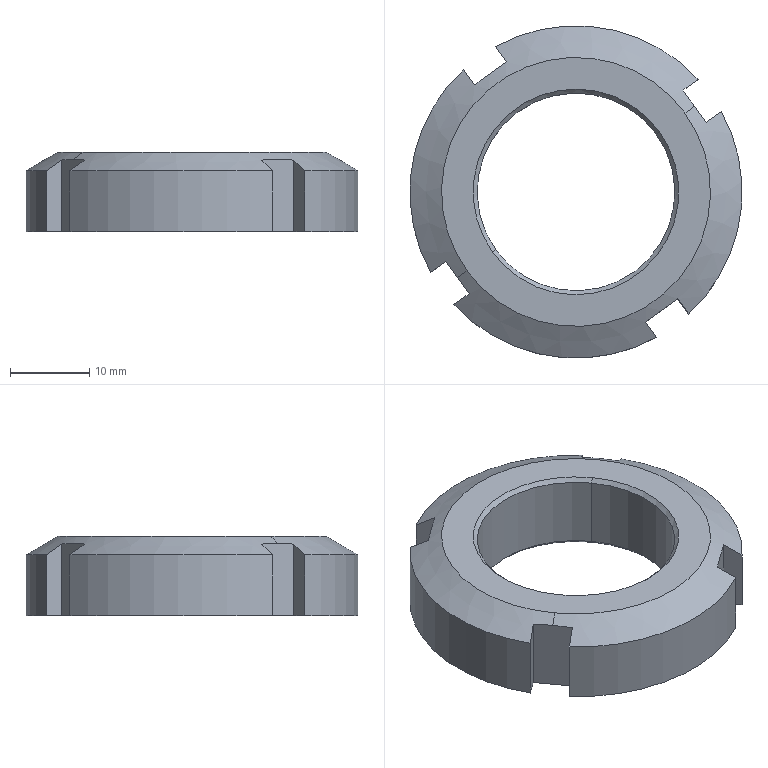Component | SolidWorks | M25_1.5RoundNut(GB-T812-1988)0-2 | 1 solid | 26 faces | box 42 x 42 x 10 mm | volume 7943 mm3 | plane 14 | cone 6 | cylinder 6 | commonest cylinder face diameters 42 x4 25 x2
build123d program:
from build123d import *

# Parameters (mm, degrees)
SKETCH2_W          = 5
SKETCH2_H          = 4.32
SKETCH2_W_2        = 4.32
SKETCH2_H_2        = 5
CUT_EXTRUDE1_DEPTH = 32.337


with BuildPart() as part:
    # Sketch1 → Revolve1 (revolve)
    with BuildSketch(Plane.XY, mode=Mode.PRIVATE) as revolve1_sk:
        Polygon((17, 5), (21, 2.69), (21, -5), (13, -5), (12.5, -4.5), (12.5, 4.5), (13, 5), align=None)
    revolve(revolve1_sk.sketch.rotate(Axis((0, 38.731, 0), (0, -1, 0)), 90), axis=Axis((0, 38.731, 0), (0, -1, 0)))

    # Sketch2 → Cut-Extrude1 (cut, through all)
    with BuildSketch(Plane(origin=(0, 5, 0), x_dir=(1, 0, 0), z_dir=(0, 1, 0))):
        with Locations((0, 20.66)):
            Rectangle(SKETCH2_W, SKETCH2_H)
        with Locations((20.66, 0)):
            Rectangle(SKETCH2_W_2, SKETCH2_H_2)
        with Locations((0, -20.66)):
            Rectangle(SKETCH2_W, SKETCH2_H)
        with Locations((-20.66, 0)):
            Rectangle(SKETCH2_W_2, SKETCH2_H_2)
    extrude(amount=-CUT_EXTRUDE1_DEPTH, mode=Mode.SUBTRACT)


solid = part.part

# Placed as in the assembly
solid = solid.moved(Location((-15.093, -37.782, 199.255), (-90, -35.881, -180)))
STEP:
#1=COLOUR_RGB('',0.7922,0.8196,0.9333);
#2=FILL_AREA_STYLE_COLOUR('',#1);
#3=FILL_AREA_STYLE('',(#2));
#4=SURFACE_STYLE_FILL_AREA(#3);
#5=SURFACE_SIDE_STYLE('',(#4));
#6=SURFACE_STYLE_USAGE(.BOTH.,#5);
#7=PRESENTATION_STYLE_ASSIGNMENT((#6));
#8=CARTESIAN_POINT('',(-0.1955,-1.199,7.668));
#9=VERTEX_POINT('',#8);
#10=CARTESIAN_POINT('',(-0.993,-1.776,7.668));
#11=VERTEX_POINT('',#10);
#12=CARTESIAN_POINT('',(-0.5942,-1.487,7.668));
#13=DIRECTION('',(0.,0.,1.));
#14=DIRECTION('',(-0.8102,-0.5861,0.));
#15=AXIS2_PLACEMENT_3D('',#12,#13,#14);
#16=CIRCLE('',#15,0.4921);
#17=EDGE_CURVE('',#9,#11,#16,.T.);
#18=ORIENTED_EDGE('',*,*,#17,.T.);
#19=CARTESIAN_POINT('',(-1.009,-1.787,7.648));
#20=VERTEX_POINT('',#19);
#21=CARTESIAN_POINT('',(-0.993,-1.776,7.668));
#22=DIRECTION('',(-0.5729,-0.4144,-0.7071));
#23=VECTOR('',#22,39.37);
#24=LINE('',#21,#23);
#25=EDGE_CURVE('',#11,#20,#24,.T.);
#26=ORIENTED_EDGE('',*,*,#25,.T.);
#27=CARTESIAN_POINT('',(-0.1795,-1.187,7.648));
#28=VERTEX_POINT('',#27);
#29=CARTESIAN_POINT('',(-0.5942,-1.487,7.648));
#30=DIRECTION('',(0.,0.,1.));
#31=DIRECTION('',(-0.8102,-0.5861,0.));
#32=AXIS2_PLACEMENT_3D('',#29,#30,#31);
#33=CIRCLE('',#32,0.5118);
#34=EDGE_CURVE('',#28,#20,#33,.T.);
#35=ORIENTED_EDGE('',*,*,#34,.F.);
#36=CARTESIAN_POINT('',(-0.1955,-1.199,7.668));
#37=DIRECTION('',(0.5729,0.4144,-0.7071));
#38=VECTOR('',#37,39.37);
#39=LINE('',#36,#38);
#40=EDGE_CURVE('',#9,#28,#39,.T.);
#41=ORIENTED_EDGE('',*,*,#40,.F.);
#42=EDGE_LOOP('',(#18,#26,#35,#41));
#43=FACE_OUTER_BOUND('',#42,.T.);
#44=CARTESIAN_POINT('',(-0.5942,-1.487,7.668));
#45=DIRECTION('',(-0.,-0.,-1.));
#46=DIRECTION('',(0.8102,0.5861,0.));
#47=AXIS2_PLACEMENT_3D('',#44,#45,#46);
#48=CONICAL_SURFACE('',#47,0.4921,0.7854);
#49=ADVANCED_FACE('',(#43),#48,.F.);
#50=ORIENTED_EDGE('',*,*,#17,.F.);
#51=CARTESIAN_POINT('',(-0.1955,-1.199,8.022));
#52=VERTEX_POINT('',#51);
#53=CARTESIAN_POINT('',(-0.1955,-1.199,9.37));
#54=DIRECTION('',(0.,0.,1.));
#55=VECTOR('',#54,39.37);
#56=LINE('',#53,#55);
#57=EDGE_CURVE('',#9,#52,#56,.T.);
#58=ORIENTED_EDGE('',*,*,#57,.T.);
#59=CARTESIAN_POINT('',(-0.993,-1.776,8.022));
#60=VERTEX_POINT('',#59);
#61=CARTESIAN_POINT('',(-0.5942,-1.487,8.022));
#62=DIRECTION('',(0.,0.,1.));
#63=DIRECTION('',(-0.8102,-0.5861,0.));
#64=AXIS2_PLACEMENT_3D('',#61,#62,#63);
#65=CIRCLE('',#64,0.4921);
#66=EDGE_CURVE('',#52,#60,#65,.T.);
#67=ORIENTED_EDGE('',*,*,#66,.T.);
#68=CARTESIAN_POINT('',(-0.993,-1.776,9.37));
#69=DIRECTION('',(0.,0.,1.));
#70=VECTOR('',#69,39.37);
#71=LINE('',#68,#70);
#72=EDGE_CURVE('',#11,#60,#71,.T.);
#73=ORIENTED_EDGE('',*,*,#72,.F.);
#74=EDGE_LOOP('',(#50,#58,#67,#73));
#75=FACE_OUTER_BOUND('',#74,.T.);
#76=CARTESIAN_POINT('',(-0.5942,-1.487,9.37));
#77=DIRECTION('',(0.,0.,1.));
#78=DIRECTION('',(-0.8102,-0.5861,0.));
#79=AXIS2_PLACEMENT_3D('',#76,#77,#78);
#80=CYLINDRICAL_SURFACE('',#79,0.4921);
#81=ADVANCED_FACE('',(#75),#80,.F.);
#82=ORIENTED_EDGE('',*,*,#66,.F.);
#83=CARTESIAN_POINT('',(-0.1795,-1.187,8.042));
#84=VERTEX_POINT('',#83);
#85=CARTESIAN_POINT('',(-0.1795,-1.187,8.042));
#86=DIRECTION('',(0.5729,0.4144,0.7071));
#87=VECTOR('',#86,39.37);
#88=LINE('',#85,#87);
#89=EDGE_CURVE('',#52,#84,#88,.T.);
#90=ORIENTED_EDGE('',*,*,#89,.T.);
#91=CARTESIAN_POINT('',(-1.009,-1.787,8.042));
#92=VERTEX_POINT('',#91);
#93=CARTESIAN_POINT('',(-0.5942,-1.487,8.042));
#94=DIRECTION('',(0.,0.,1.));
#95=DIRECTION('',(-0.8102,-0.5861,0.));
#96=AXIS2_PLACEMENT_3D('',#93,#94,#95);
#97=CIRCLE('',#96,0.5118);
#98=EDGE_CURVE('',#84,#92,#97,.T.);
#99=ORIENTED_EDGE('',*,*,#98,.T.);
#100=CARTESIAN_POINT('',(-1.009,-1.787,8.042));
#101=DIRECTION('',(-0.5729,-0.4144,0.7071));
#102=VECTOR('',#101,39.37);
#103=LINE('',#100,#102);
#104=EDGE_CURVE('',#60,#92,#103,.T.);
#105=ORIENTED_EDGE('',*,*,#104,.F.);
#106=EDGE_LOOP('',(#82,#90,#99,#105));
#107=FACE_OUTER_BOUND('',#106,.T.);
#108=CARTESIAN_POINT('',(-0.5942,-1.487,8.042));
#109=DIRECTION('',(0.,0.,1.));
#110=DIRECTION('',(-0.8102,-0.5861,0.));
#111=AXIS2_PLACEMENT_3D('',#108,#109,#110);
#112=CONICAL_SURFACE('',#111,0.5118,0.7854);
#113=ADVANCED_FACE('',(#107),#112,.F.);
#114=CARTESIAN_POINT('',(-1.137,-1.88,8.042));
#115=VERTEX_POINT('',#114);
#116=CARTESIAN_POINT('',(-0.05193,-1.095,8.042));
#117=VERTEX_POINT('',#116);
#118=CARTESIAN_POINT('',(-0.5942,-1.487,8.042));
#119=DIRECTION('',(0.,0.,1.));
#120=DIRECTION('',(-0.8102,-0.5861,0.));
#121=AXIS2_PLACEMENT_3D('',#118,#119,#120);
#122=CIRCLE('',#121,0.6693);
#123=EDGE_CURVE('',#115,#117,#122,.T.);
#124=ORIENTED_EDGE('',*,*,#123,.F.);
#125=CARTESIAN_POINT('',(-1.184,-1.914,8.007));
#126=VERTEX_POINT('',#125);
#127=CARTESIAN_POINT('',(-1.264,-1.972,7.951));
#128=DIRECTION('',(-0.7016,-0.5075,-0.5001));
#129=VECTOR('',#128,39.37);
#130=LINE('',#127,#129);
#131=EDGE_CURVE('',#115,#126,#130,.T.);
#132=ORIENTED_EDGE('',*,*,#131,.T.);
#133=CARTESIAN_POINT('',(-1.127,-1.994,8.004));
#134=VERTEX_POINT('',#133);
#135=CARTESIAN_POINT('',(-1.184,-1.914,8.007));
#136=CARTESIAN_POINT('',(-1.165,-1.941,8.007));
#137=CARTESIAN_POINT('',(-1.146,-1.968,8.006));
#138=CARTESIAN_POINT('',(-1.127,-1.994,8.004));
#139=B_SPLINE_CURVE_WITH_KNOTS('',3,(#135,#136,#137,#138),.UNSPECIFIED.,.F.,.F.,(4,4),(0.01295,0.01546),.UNSPECIFIED.);
#140=EDGE_CURVE('',#126,#134,#139,.T.);
#141=ORIENTED_EDGE('',*,*,#140,.T.);
#142=CARTESIAN_POINT('',(-1.202,-2.048,7.951));
#143=VERTEX_POINT('',#142);
#144=CARTESIAN_POINT('',(-1.127,-1.994,8.004));
#145=CARTESIAN_POINT('',(-1.152,-2.012,7.986));
#146=CARTESIAN_POINT('',(-1.177,-2.03,7.968));
#147=CARTESIAN_POINT('',(-1.202,-2.048,7.951));
#148=B_SPLINE_CURVE_WITH_KNOTS('',3,(#144,#145,#146,#147),.UNSPECIFIED.,.F.,.F.,(4,4),(0.005721,0.00843),.UNSPECIFIED.);
#149=EDGE_CURVE('',#134,#143,#148,.T.);
#150=ORIENTED_EDGE('',*,*,#149,.T.);
#151=CARTESIAN_POINT('',(-0.1928,-2.21,7.951));
#152=VERTEX_POINT('',#151);
#153=CARTESIAN_POINT('',(-0.5942,-1.487,7.951));
#154=DIRECTION('',(0.,0.,1.));
#155=DIRECTION('',(-0.8102,-0.5861,0.));
#156=AXIS2_PLACEMENT_3D('',#153,#154,#155);
#157=CIRCLE('',#156,0.8268);
#158=EDGE_CURVE('',#143,#152,#157,.T.);
#159=ORIENTED_EDGE('',*,*,#158,.T.);
#160=CARTESIAN_POINT('',(-0.2471,-2.135,8.004));
#161=VERTEX_POINT('',#160);
#162=CARTESIAN_POINT('',(-0.1928,-2.21,7.951));
#163=CARTESIAN_POINT('',(-0.2109,-2.185,7.968));
#164=CARTESIAN_POINT('',(-0.229,-2.16,7.986));
#165=CARTESIAN_POINT('',(-0.2471,-2.135,8.004));
#166=B_SPLINE_CURVE_WITH_KNOTS('',3,(#162,#163,#164,#165),.UNSPECIFIED.,.F.,.F.,(4,4),(0.004032,0.006741),.UNSPECIFIED.);
#167=EDGE_CURVE('',#152,#161,#166,.T.);
#168=ORIENTED_EDGE('',*,*,#167,.T.);
#169=CARTESIAN_POINT('',(-0.08759,-2.02,8.004));
#170=VERTEX_POINT('',#169);
#171=CARTESIAN_POINT('',(-0.2471,-2.135,8.004));
#172=CARTESIAN_POINT('',(-0.2207,-2.116,8.006));
#173=CARTESIAN_POINT('',(-0.1942,-2.097,8.007));
#174=CARTESIAN_POINT('',(-0.1411,-2.059,8.007));
#175=CARTESIAN_POINT('',(-0.1142,-2.039,8.006));
#176=CARTESIAN_POINT('',(-0.08759,-2.02,8.004));
#177=B_SPLINE_CURVE_WITH_KNOTS('',3,(#171,#172,#173,#174,#175,#176),.UNSPECIFIED.,.F.,.F.,(4,2,4),(0.00681,0.009296,0.01178),.UNSPECIFIED.);
#178=EDGE_CURVE('',#161,#170,#177,.T.);
#179=ORIENTED_EDGE('',*,*,#178,.T.);
#180=CARTESIAN_POINT('',(-0.03335,-2.095,7.951));
#181=VERTEX_POINT('',#180);
#182=CARTESIAN_POINT('',(-0.08759,-2.02,8.004));
#183=CARTESIAN_POINT('',(-0.06951,-2.045,7.986));
#184=CARTESIAN_POINT('',(-0.05143,-2.07,7.968));
#185=CARTESIAN_POINT('',(-0.03335,-2.095,7.951));
#186=B_SPLINE_CURVE_WITH_KNOTS('',3,(#182,#183,#184,#185),.UNSPECIFIED.,.F.,.F.,(4,4),(0.005721,0.00843),.UNSPECIFIED.);
#187=EDGE_CURVE('',#170,#181,#186,.T.);
#188=ORIENTED_EDGE('',*,*,#187,.T.);
#189=CARTESIAN_POINT('',(0.1286,-1.086,7.951));
#190=VERTEX_POINT('',#189);
#191=CARTESIAN_POINT('',(-0.5942,-1.487,7.951));
#192=DIRECTION('',(0.,0.,1.));
#193=DIRECTION('',(-0.8102,-0.5861,0.));
#194=AXIS2_PLACEMENT_3D('',#191,#192,#193);
#195=CIRCLE('',#194,0.8268);
#196=EDGE_CURVE('',#181,#190,#195,.T.);
#197=ORIENTED_EDGE('',*,*,#196,.T.);
#198=CARTESIAN_POINT('',(0.0536,-1.14,8.004));
#199=VERTEX_POINT('',#198);
#200=CARTESIAN_POINT('',(0.1286,-1.086,7.951));
#201=CARTESIAN_POINT('',(0.126,-1.088,7.952));
#202=CARTESIAN_POINT('',(0.1233,-1.09,7.954));
#203=CARTESIAN_POINT('',(0.1207,-1.092,7.956));
#204=CARTESIAN_POINT('',(0.09834,-1.108,7.972));
#205=CARTESIAN_POINT('',(0.07597,-1.124,7.988));
#206=CARTESIAN_POINT('',(0.0536,-1.14,8.004));
#207=B_SPLINE_CURVE_WITH_KNOTS('',3,(#200,#201,#202,#203,#204,#205,#206),.UNSPECIFIED.,.F.,.F.,(4,3,4),(0.005946,0.006231,0.008655),.UNSPECIFIED.);
#208=EDGE_CURVE('',#190,#199,#207,.T.);
#209=ORIENTED_EDGE('',*,*,#208,.T.);
#210=CARTESIAN_POINT('',(-0.004084,-1.061,8.007));
#211=VERTEX_POINT('',#210);
#212=CARTESIAN_POINT('',(0.0536,-1.14,8.004));
#213=CARTESIAN_POINT('',(0.03445,-1.114,8.006));
#214=CARTESIAN_POINT('',(0.01523,-1.087,8.007));
#215=CARTESIAN_POINT('',(-0.004084,-1.061,8.007));
#216=B_SPLINE_CURVE_WITH_KNOTS('',3,(#212,#213,#214,#215),.UNSPECIFIED.,.F.,.F.,(4,4),(0.00681,0.009305),.UNSPECIFIED.);
#217=EDGE_CURVE('',#199,#211,#216,.T.);
#218=ORIENTED_EDGE('',*,*,#217,.T.);
#219=CARTESIAN_POINT('',(0.07566,-1.003,7.951));
#220=DIRECTION('',(0.7016,0.5075,-0.5001));
#221=VECTOR('',#220,39.37);
#222=LINE('',#219,#221);
#223=EDGE_CURVE('',#117,#211,#222,.T.);
#224=ORIENTED_EDGE('',*,*,#223,.F.);
#225=EDGE_LOOP('',(#124,#132,#141,#150,#159,#168,#179,#188,#197,#209,#218,#224));
#226=FACE_OUTER_BOUND('',#225,.T.);
#227=CARTESIAN_POINT('',(-0.5942,-1.487,7.951));
#228=DIRECTION('',(-0.,-0.,-1.));
#229=DIRECTION('',(0.8102,0.5861,0.));
#230=AXIS2_PLACEMENT_3D('',#227,#228,#229);
#231=CONICAL_SURFACE('',#230,0.8268,1.047);
#232=ADVANCED_FACE('',(#226),#231,.T.);
#233=CARTESIAN_POINT('',(-1.202,-2.048,7.648));
#234=VERTEX_POINT('',#233);
#235=CARTESIAN_POINT('',(-0.1928,-2.21,7.648));
#236=VERTEX_POINT('',#235);
#237=CARTESIAN_POINT('',(-0.5942,-1.487,7.648));
#238=DIRECTION('',(0.,0.,1.));
#239=DIRECTION('',(-0.8102,-0.5861,0.));
#240=AXIS2_PLACEMENT_3D('',#237,#238,#239);
#241=CIRCLE('',#240,0.8268);
#242=EDGE_CURVE('',#234,#236,#241,.T.);
#243=ORIENTED_EDGE('',*,*,#242,.T.);
#244=CARTESIAN_POINT('',(-0.1928,-2.21,9.37));
#245=DIRECTION('',(0.,0.,1.));
#246=VECTOR('',#245,39.37);
#247=LINE('',#244,#246);
#248=EDGE_CURVE('',#236,#152,#247,.T.);
#249=ORIENTED_EDGE('',*,*,#248,.T.);
#250=ORIENTED_EDGE('',*,*,#158,.F.);
#251=CARTESIAN_POINT('',(-1.202,-2.048,9.37));
#252=DIRECTION('',(-0.,-0.,-1.));
#253=VECTOR('',#252,39.37);
#254=LINE('',#251,#253);
#255=EDGE_CURVE('',#143,#234,#254,.T.);
#256=ORIENTED_EDGE('',*,*,#255,.T.);
#257=EDGE_LOOP('',(#243,#249,#250,#256));
#258=FACE_OUTER_BOUND('',#257,.T.);
#259=CARTESIAN_POINT('',(-0.5942,-1.487,9.37));
#260=DIRECTION('',(0.,0.,1.));
#261=DIRECTION('',(-0.8102,-0.5861,0.));
#262=AXIS2_PLACEMENT_3D('',#259,#260,#261);
#263=CYLINDRICAL_SURFACE('',#262,0.8268);
#264=ADVANCED_FACE('',(#258),#263,.T.);
#265=CARTESIAN_POINT('',(-1.155,-0.88,7.648));
#266=VERTEX_POINT('',#265);
#267=CARTESIAN_POINT('',(-1.317,-1.889,7.648));
#268=VERTEX_POINT('',#267);
#269=CARTESIAN_POINT('',(-0.5942,-1.487,7.648));
#270=DIRECTION('',(0.,0.,1.));
#271=DIRECTION('',(-0.8102,-0.5861,0.));
#272=AXIS2_PLACEMENT_3D('',#269,#270,#271);
#273=CIRCLE('',#272,0.8268);
#274=EDGE_CURVE('',#266,#268,#273,.T.);
#275=ORIENTED_EDGE('',*,*,#274,.T.);
#276=CARTESIAN_POINT('',(-1.317,-1.889,7.951));
#277=VERTEX_POINT('',#276);
#278=CARTESIAN_POINT('',(-1.317,-1.889,9.37));
#279=DIRECTION('',(0.,0.,1.));
#280=VECTOR('',#279,39.37);
#281=LINE('',#278,#280);
#282=EDGE_CURVE('',#268,#277,#281,.T.);
#283=ORIENTED_EDGE('',*,*,#282,.T.);
#284=CARTESIAN_POINT('',(-1.155,-0.88,7.951));
#285=VERTEX_POINT('',#284);
#286=CARTESIAN_POINT('',(-0.5942,-1.487,7.951));
#287=DIRECTION('',(0.,0.,1.));
#288=DIRECTION('',(-0.8102,-0.5861,0.));
#289=AXIS2_PLACEMENT_3D('',#286,#287,#288);
#290=CIRCLE('',#289,0.8268);
#291=EDGE_CURVE('',#285,#277,#290,.T.);
#292=ORIENTED_EDGE('',*,*,#291,.F.);
#293=CARTESIAN_POINT('',(-1.155,-0.88,9.37));
#294=DIRECTION('',(-0.,-0.,-1.));
#295=VECTOR('',#294,39.37);
#296=LINE('',#293,#295);
#297=EDGE_CURVE('',#285,#266,#296,.T.);
#298=ORIENTED_EDGE('',*,*,#297,.T.);
#299=EDGE_LOOP('',(#275,#283,#292,#298));
#300=FACE_OUTER_BOUND('',#299,.T.);
#301=CARTESIAN_POINT('',(-0.5942,-1.487,9.37));
#302=DIRECTION('',(0.,0.,1.));
#303=DIRECTION('',(-0.8102,-0.5861,0.));
#304=AXIS2_PLACEMENT_3D('',#301,#302,#303);
#305=CYLINDRICAL_SURFACE('',#304,0.8268);
#306=ADVANCED_FACE('',(#300),#305,.T.);
#307=CARTESIAN_POINT('',(0.01321,-0.9266,7.648));
#308=VERTEX_POINT('',#307);
#309=CARTESIAN_POINT('',(-0.9956,-0.7647,7.648));
#310=VERTEX_POINT('',#309);
#311=CARTESIAN_POINT('',(-0.5942,-1.487,7.648));
#312=DIRECTION('',(0.,0.,1.));
#313=DIRECTION('',(-0.8102,-0.5861,0.));
#314=AXIS2_PLACEMENT_3D('',#311,#312,#313);
#315=CIRCLE('',#314,0.8268);
#316=EDGE_CURVE('',#308,#310,#315,.T.);
#317=ORIENTED_EDGE('',*,*,#316,.T.);
#318=CARTESIAN_POINT('',(-0.9956,-0.7647,7.951));
#319=VERTEX_POINT('',#318);
#320=CARTESIAN_POINT('',(-0.9956,-0.7647,9.37));
#321=DIRECTION('',(0.,0.,1.));
#322=VECTOR('',#321,39.37);
#323=LINE('',#320,#322);
#324=EDGE_CURVE('',#310,#319,#323,.T.);
#325=ORIENTED_EDGE('',*,*,#324,.T.);
#326=CARTESIAN_POINT('',(0.01321,-0.9266,7.951));
#327=VERTEX_POINT('',#326);
#328=CARTESIAN_POINT('',(-0.5942,-1.487,7.951));
#329=DIRECTION('',(0.,0.,1.));
#330=DIRECTION('',(-0.8102,-0.5861,0.));
#331=AXIS2_PLACEMENT_3D('',#328,#329,#330);
#332=CIRCLE('',#331,0.8268);
#333=EDGE_CURVE('',#327,#319,#332,.T.);
#334=ORIENTED_EDGE('',*,*,#333,.F.);
#335=CARTESIAN_POINT('',(0.01321,-0.9266,9.37));
#336=DIRECTION('',(-0.,-0.,-1.));
#337=VECTOR('',#336,39.37);
#338=LINE('',#335,#337);
#339=EDGE_CURVE('',#327,#308,#338,.T.);
#340=ORIENTED_EDGE('',*,*,#339,.T.);
#341=EDGE_LOOP('',(#317,#325,#334,#340));
#342=FACE_OUTER_BOUND('',#341,.T.);
#343=CARTESIAN_POINT('',(-0.5942,-1.487,9.37));
#344=DIRECTION('',(0.,0.,1.));
#345=DIRECTION('',(-0.8102,-0.5861,0.));
#346=AXIS2_PLACEMENT_3D('',#343,#344,#345);
#347=CYLINDRICAL_SURFACE('',#346,0.8268);
#348=ADVANCED_FACE('',(#342),#347,.T.);
#349=ORIENTED_EDGE('',*,*,#196,.F.);
#350=CARTESIAN_POINT('',(-0.03335,-2.095,7.648));
#351=VERTEX_POINT('',#350);
#352=CARTESIAN_POINT('',(-0.03335,-2.095,9.37));
#353=DIRECTION('',(-0.,-0.,-1.));
#354=VECTOR('',#353,39.37);
#355=LINE('',#352,#354);
#356=EDGE_CURVE('',#181,#351,#355,.T.);
#357=ORIENTED_EDGE('',*,*,#356,.T.);
#358=CARTESIAN_POINT('',(0.1286,-1.086,7.648));
#359=VERTEX_POINT('',#358);
#360=CARTESIAN_POINT('',(-0.5942,-1.487,7.648));
#361=DIRECTION('',(0.,0.,1.));
#362=DIRECTION('',(-0.8102,-0.5861,0.));
#363=AXIS2_PLACEMENT_3D('',#360,#361,#362);
#364=CIRCLE('',#363,0.8268);
#365=EDGE_CURVE('',#351,#359,#364,.T.);
#366=ORIENTED_EDGE('',*,*,#365,.T.);
#367=CARTESIAN_POINT('',(0.1286,-1.086,9.37));
#368=DIRECTION('',(0.,0.,1.));
#369=VECTOR('',#368,39.37);
#370=LINE('',#367,#369);
#371=EDGE_CURVE('',#359,#190,#370,.T.);
#372=ORIENTED_EDGE('',*,*,#371,.T.);
#373=EDGE_LOOP('',(#349,#357,#366,#372));
#374=FACE_OUTER_BOUND('',#373,.T.);
#375=CARTESIAN_POINT('',(-0.5942,-1.487,9.37));
#376=DIRECTION('',(0.,0.,1.));
#377=DIRECTION('',(-0.8102,-0.5861,0.));
#378=AXIS2_PLACEMENT_3D('',#375,#376,#377);
#379=CYLINDRICAL_SURFACE('',#378,0.8268);
#380=ADVANCED_FACE('',(#374),#379,.T.);
#381=ORIENTED_EDGE('',*,*,#131,.F.);
#382=CARTESIAN_POINT('',(-0.5942,-1.487,8.042));
#383=DIRECTION('',(0.,0.,1.));
#384=DIRECTION('',(-0.8102,-0.5861,0.));
#385=AXIS2_PLACEMENT_3D('',#382,#383,#384);
#386=CIRCLE('',#385,0.6693);
#387=EDGE_CURVE('',#117,#115,#386,.T.);
#388=ORIENTED_EDGE('',*,*,#387,.F.);
#389=ORIENTED_EDGE('',*,*,#223,.T.);
#390=CARTESIAN_POINT('',(-0.06177,-0.9808,8.004));
#391=VERTEX_POINT('',#390);
#392=CARTESIAN_POINT('',(-0.004084,-1.061,8.007));
#393=CARTESIAN_POINT('',(-0.02325,-1.034,8.007));
#394=CARTESIAN_POINT('',(-0.04256,-1.007,8.006));
#395=CARTESIAN_POINT('',(-0.06177,-0.9808,8.004));
#396=B_SPLINE_CURVE_WITH_KNOTS('',3,(#392,#393,#394,#395),.UNSPECIFIED.,.F.,.F.,(4,4),(0.009305,0.01178),.UNSPECIFIED.);
#397=EDGE_CURVE('',#211,#391,#396,.T.);
#398=ORIENTED_EDGE('',*,*,#397,.T.);
#399=CARTESIAN_POINT('',(-0.06177,-0.9808,8.004));
#400=CARTESIAN_POINT('',(-0.0394,-0.9647,7.988));
#401=CARTESIAN_POINT('',(-0.01704,-0.9485,7.972));
#402=CARTESIAN_POINT('',(0.005322,-0.9323,7.956));
#403=CARTESIAN_POINT('',(0.007953,-0.9304,7.954));
#404=CARTESIAN_POINT('',(0.01058,-0.9285,7.952));
#405=CARTESIAN_POINT('',(0.01321,-0.9266,7.951));
#406=B_SPLINE_CURVE_WITH_KNOTS('',3,(#399,#400,#401,#402,#403,#404,#405),.UNSPECIFIED.,.F.,.F.,(4,3,4),(0.003807,0.006231,0.006516),.UNSPECIFIED.);
#407=EDGE_CURVE('',#391,#327,#406,.T.);
#408=ORIENTED_EDGE('',*,*,#407,.T.);
#409=ORIENTED_EDGE('',*,*,#333,.T.);
#410=CARTESIAN_POINT('',(-0.9414,-0.8396,8.004));
#411=VERTEX_POINT('',#410);
#412=CARTESIAN_POINT('',(-0.9956,-0.7647,7.951));
#413=CARTESIAN_POINT('',(-0.9937,-0.7673,7.952));
#414=CARTESIAN_POINT('',(-0.9918,-0.7699,7.954));
#415=CARTESIAN_POINT('',(-0.9899,-0.7725,7.956));
#416=CARTESIAN_POINT('',(-0.9737,-0.7949,7.972));
#417=CARTESIAN_POINT('',(-0.9575,-0.8173,7.988));
#418=CARTESIAN_POINT('',(-0.9414,-0.8396,8.004));
#419=B_SPLINE_CURVE_WITH_KNOTS('',3,(#412,#413,#414,#415,#416,#417,#418),.UNSPECIFIED.,.F.,.F.,(4,3,4),(0.005946,0.006231,0.008655),.UNSPECIFIED.);
#420=EDGE_CURVE('',#319,#411,#419,.T.);
#421=ORIENTED_EDGE('',*,*,#420,.T.);
#422=CARTESIAN_POINT('',(-1.101,-0.955,8.004));
#423=VERTEX_POINT('',#422);
#424=CARTESIAN_POINT('',(-0.9414,-0.8396,8.004));
#425=CARTESIAN_POINT('',(-0.968,-0.8589,8.006));
#426=CARTESIAN_POINT('',(-0.9948,-0.8783,8.007));
#427=CARTESIAN_POINT('',(-1.048,-0.9168,8.007));
#428=CARTESIAN_POINT('',(-1.074,-0.9359,8.006));
#429=CARTESIAN_POINT('',(-1.101,-0.955,8.004));
#430=B_SPLINE_CURVE_WITH_KNOTS('',3,(#424,#425,#426,#427,#428,#429),.UNSPECIFIED.,.F.,.F.,(4,2,4),(0.01047,0.01296,0.01546),.UNSPECIFIED.);
#431=EDGE_CURVE('',#411,#423,#430,.T.);
#432=ORIENTED_EDGE('',*,*,#431,.T.);
#433=CARTESIAN_POINT('',(-1.101,-0.955,8.004));
#434=CARTESIAN_POINT('',(-1.117,-0.9326,7.988));
#435=CARTESIAN_POINT('',(-1.133,-0.9103,7.972));
#436=CARTESIAN_POINT('',(-1.149,-0.8879,7.956));
#437=CARTESIAN_POINT('',(-1.151,-0.8853,7.954));
#438=CARTESIAN_POINT('',(-1.153,-0.8827,7.952));
#439=CARTESIAN_POINT('',(-1.155,-0.88,7.951));
#440=B_SPLINE_CURVE_WITH_KNOTS('',3,(#433,#434,#435,#436,#437,#438,#439),.UNSPECIFIED.,.F.,.F.,(4,3,4),(0.003807,0.006231,0.006516),.UNSPECIFIED.);
#441=EDGE_CURVE('',#423,#285,#440,.T.);
#442=ORIENTED_EDGE('',*,*,#441,.T.);
#443=ORIENTED_EDGE('',*,*,#291,.T.);
#444=CARTESIAN_POINT('',(-1.242,-1.835,8.004));
#445=VERTEX_POINT('',#444);
#446=CARTESIAN_POINT('',(-1.317,-1.889,7.951));
#447=CARTESIAN_POINT('',(-1.292,-1.871,7.968));
#448=CARTESIAN_POINT('',(-1.267,-1.853,7.986));
#449=CARTESIAN_POINT('',(-1.242,-1.835,8.004));
#450=B_SPLINE_CURVE_WITH_KNOTS('',3,(#446,#447,#448,#449),.UNSPECIFIED.,.F.,.F.,(4,4),(0.004032,0.006741),.UNSPECIFIED.);
#451=EDGE_CURVE('',#277,#445,#450,.T.);
#452=ORIENTED_EDGE('',*,*,#451,.T.);
#453=CARTESIAN_POINT('',(-1.242,-1.835,8.004));
#454=CARTESIAN_POINT('',(-1.223,-1.861,8.006));
#455=CARTESIAN_POINT('',(-1.204,-1.888,8.007));
#456=CARTESIAN_POINT('',(-1.184,-1.914,8.007));
#457=B_SPLINE_CURVE_WITH_KNOTS('',3,(#453,#454,#455,#456),.UNSPECIFIED.,.F.,.F.,(4,4),(0.01047,0.01295),.UNSPECIFIED.);
#458=EDGE_CURVE('',#445,#126,#457,.T.);
#459=ORIENTED_EDGE('',*,*,#458,.T.);
#460=EDGE_LOOP('',(#381,#388,#389,#398,#408,#409,#421,#432,#442,#443,#452,#459));
#461=FACE_OUTER_BOUND('',#460,.T.);
#462=CARTESIAN_POINT('',(-0.5942,-1.487,7.951));
#463=DIRECTION('',(-0.,-0.,-1.));
#464=DIRECTION('',(0.8102,0.5861,0.));
#465=AXIS2_PLACEMENT_3D('',#462,#463,#464);
#466=CONICAL_SURFACE('',#465,0.8268,1.047);
#467=ADVANCED_FACE('',(#461),#466,.T.);
#468=CARTESIAN_POINT('',(-0.5942,-1.487,8.042));
#469=DIRECTION('',(0.,0.,1.));
#470=DIRECTION('',(-0.8102,-0.5861,0.));
#471=AXIS2_PLACEMENT_3D('',#468,#469,#470);
#472=CIRCLE('',#471,0.5118);
#473=EDGE_CURVE('',#92,#84,#472,.T.);
#474=ORIENTED_EDGE('',*,*,#473,.F.);
#475=ORIENTED_EDGE('',*,*,#98,.F.);
#476=EDGE_LOOP('',(#474,#475));
#477=FACE_BOUND('',#476,.T.);
#478=ORIENTED_EDGE('',*,*,#387,.T.);
#479=ORIENTED_EDGE('',*,*,#123,.T.);
#480=EDGE_LOOP('',(#478,#479));
#481=FACE_OUTER_BOUND('',#480,.T.);
#482=CARTESIAN_POINT('',(-0.2942,-1.902,8.042));
#483=DIRECTION('',(-0.,-0.,-1.));
#484=DIRECTION('',(0.8102,0.5861,-0.));
#485=AXIS2_PLACEMENT_3D('',#482,#483,#484);
#486=PLANE('',#485);
#487=ADVANCED_FACE('',(#477,#481),#486,.F.);
#488=ORIENTED_EDGE('',*,*,#89,.F.);
#489=CARTESIAN_POINT('',(-0.5942,-1.487,8.022));
#490=DIRECTION('',(0.,0.,1.));
#491=DIRECTION('',(-0.8102,-0.5861,0.));
#492=AXIS2_PLACEMENT_3D('',#489,#490,#491);
#493=CIRCLE('',#492,0.4921);
#494=EDGE_CURVE('',#60,#52,#493,.T.);
#495=ORIENTED_EDGE('',*,*,#494,.F.);
#496=ORIENTED_EDGE('',*,*,#104,.T.);
#497=ORIENTED_EDGE('',*,*,#473,.T.);
#498=EDGE_LOOP('',(#488,#495,#496,#497));
#499=FACE_OUTER_BOUND('',#498,.T.);
#500=CARTESIAN_POINT('',(-0.5942,-1.487,8.042));
#501=DIRECTION('',(0.,0.,1.));
#502=DIRECTION('',(-0.8102,-0.5861,0.));
#503=AXIS2_PLACEMENT_3D('',#500,#501,#502);
#504=CONICAL_SURFACE('',#503,0.5118,0.7854);
#505=ADVANCED_FACE('',(#499),#504,.F.);
#506=ORIENTED_EDGE('',*,*,#57,.F.);
#507=CARTESIAN_POINT('',(-0.5942,-1.487,7.668));
#508=DIRECTION('',(0.,0.,1.));
#509=DIRECTION('',(-0.8102,-0.5861,0.));
#510=AXIS2_PLACEMENT_3D('',#507,#508,#509);
#511=CIRCLE('',#510,0.4921);
#512=EDGE_CURVE('',#11,#9,#511,.T.);
#513=ORIENTED_EDGE('',*,*,#512,.F.);
#514=ORIENTED_EDGE('',*,*,#72,.T.);
#515=ORIENTED_EDGE('',*,*,#494,.T.);
#516=EDGE_LOOP('',(#506,#513,#514,#515));
#517=FACE_OUTER_BOUND('',#516,.T.);
#518=CARTESIAN_POINT('',(-0.5942,-1.487,9.37));
#519=DIRECTION('',(0.,0.,1.));
#520=DIRECTION('',(-0.8102,-0.5861,0.));
#521=AXIS2_PLACEMENT_3D('',#518,#519,#520);
#522=CYLINDRICAL_SURFACE('',#521,0.4921);
#523=ADVANCED_FACE('',(#517),#522,.F.);
#524=ORIENTED_EDGE('',*,*,#25,.F.);
#525=ORIENTED_EDGE('',*,*,#512,.T.);
#526=ORIENTED_EDGE('',*,*,#40,.T.);
#527=CARTESIAN_POINT('',(-0.5942,-1.487,7.648));
#528=DIRECTION('',(0.,0.,1.));
#529=DIRECTION('',(-0.8102,-0.5861,0.));
#530=AXIS2_PLACEMENT_3D('',#527,#528,#529);
#531=CIRCLE('',#530,0.5118);
#532=EDGE_CURVE('',#20,#28,#531,.T.);
#533=ORIENTED_EDGE('',*,*,#532,.F.);
#534=EDGE_LOOP('',(#524,#525,#526,#533));
#535=FACE_OUTER_BOUND('',#534,.T.);
#536=CARTESIAN_POINT('',(-0.5942,-1.487,7.668));
#537=DIRECTION('',(-0.,-0.,-1.));
#538=DIRECTION('',(0.8102,0.5861,0.));
#539=AXIS2_PLACEMENT_3D('',#536,#537,#538);
#540=CONICAL_SURFACE('',#539,0.4921,0.7854);
#541=ADVANCED_FACE('',(#535),#540,.F.);
#542=CARTESIAN_POINT('',(-0.08759,-2.02,7.648));
#543=VERTEX_POINT('',#542);
#544=CARTESIAN_POINT('',(-0.2471,-2.135,7.648));
#545=VERTEX_POINT('',#544);
#546=CARTESIAN_POINT('',(-0.08759,-2.02,7.648));
#547=DIRECTION('',(-0.8102,-0.5861,0.));
#548=VECTOR('',#547,39.37);
#549=LINE('',#546,#548);
#550=EDGE_CURVE('',#543,#545,#549,.T.);
#551=ORIENTED_EDGE('',*,*,#550,.T.);
#552=CARTESIAN_POINT('',(-0.1474,-2.273,7.648));
#553=DIRECTION('',(0.5861,-0.8102,0.));
#554=VECTOR('',#553,39.37);
#555=LINE('',#552,#554);
#556=EDGE_CURVE('',#545,#236,#555,.T.);
#557=ORIENTED_EDGE('',*,*,#556,.T.);
#558=ORIENTED_EDGE('',*,*,#242,.F.);
#559=CARTESIAN_POINT('',(-1.127,-1.994,7.648));
#560=VERTEX_POINT('',#559);
#561=CARTESIAN_POINT('',(-0.5365,-1.567,7.648));
#562=DIRECTION('',(0.8102,0.5861,-0.));
#563=VECTOR('',#562,39.37);
#564=LINE('',#561,#563);
#565=EDGE_CURVE('',#234,#560,#564,.T.);
#566=ORIENTED_EDGE('',*,*,#565,.T.);
#567=CARTESIAN_POINT('',(-1.242,-1.835,7.648));
#568=VERTEX_POINT('',#567);
#569=CARTESIAN_POINT('',(-1.127,-1.994,7.648));
#570=DIRECTION('',(-0.5861,0.8102,-0.));
#571=VECTOR('',#570,39.37);
#572=LINE('',#569,#571);
#573=EDGE_CURVE('',#560,#568,#572,.T.);
#574=ORIENTED_EDGE('',*,*,#573,.T.);
#575=CARTESIAN_POINT('',(-1.38,-1.934,7.648));
#576=DIRECTION('',(-0.8102,-0.5861,0.));
#577=VECTOR('',#576,39.37);
#578=LINE('',#575,#577);
#579=EDGE_CURVE('',#568,#268,#578,.T.);
#580=ORIENTED_EDGE('',*,*,#579,.T.);
#581=ORIENTED_EDGE('',*,*,#274,.F.);
#582=CARTESIAN_POINT('',(-1.101,-0.955,7.648));
#583=VERTEX_POINT('',#582);
#584=CARTESIAN_POINT('',(-0.374,-1.96,7.648));
#585=DIRECTION('',(0.5861,-0.8102,0.));
#586=VECTOR('',#585,39.37);
#587=LINE('',#584,#586);
#588=EDGE_CURVE('',#266,#583,#587,.T.);
#589=ORIENTED_EDGE('',*,*,#588,.T.);
#590=CARTESIAN_POINT('',(-0.9414,-0.8396,7.648));
#591=VERTEX_POINT('',#590);
#592=CARTESIAN_POINT('',(-1.101,-0.955,7.648));
#593=DIRECTION('',(0.8102,0.5861,-0.));
#594=VECTOR('',#593,39.37);
#595=LINE('',#592,#594);
#596=EDGE_CURVE('',#583,#591,#595,.T.);
#597=ORIENTED_EDGE('',*,*,#596,.T.);
#598=CARTESIAN_POINT('',(-1.041,-0.7018,7.648));
#599=DIRECTION('',(-0.5861,0.8102,-0.));
#600=VECTOR('',#599,39.37);
#601=LINE('',#598,#600);
#602=EDGE_CURVE('',#591,#310,#601,.T.);
#603=ORIENTED_EDGE('',*,*,#602,.T.);
#604=ORIENTED_EDGE('',*,*,#316,.F.);
#605=CARTESIAN_POINT('',(-0.06177,-0.9808,7.648));
#606=VERTEX_POINT('',#605);
#607=CARTESIAN_POINT('',(-0.6519,-1.408,7.648));
#608=DIRECTION('',(-0.8102,-0.5861,0.));
#609=VECTOR('',#608,39.37);
#610=LINE('',#607,#609);
#611=EDGE_CURVE('',#308,#606,#610,.T.);
#612=ORIENTED_EDGE('',*,*,#611,.T.);
#613=CARTESIAN_POINT('',(0.0536,-1.14,7.648));
#614=VERTEX_POINT('',#613);
#615=CARTESIAN_POINT('',(-0.06177,-0.9808,7.648));
#616=DIRECTION('',(0.5861,-0.8102,0.));
#617=VECTOR('',#616,39.37);
#618=LINE('',#615,#617);
#619=EDGE_CURVE('',#606,#614,#618,.T.);
#620=ORIENTED_EDGE('',*,*,#619,.T.);
#621=CARTESIAN_POINT('',(0.1914,-1.041,7.648));
#622=DIRECTION('',(0.8102,0.5861,-0.));
#623=VECTOR('',#622,39.37);
#624=LINE('',#621,#623);
#625=EDGE_CURVE('',#614,#359,#624,.T.);
#626=ORIENTED_EDGE('',*,*,#625,.T.);
#627=ORIENTED_EDGE('',*,*,#365,.F.);
#628=CARTESIAN_POINT('',(-0.2145,-1.844,7.648));
#629=DIRECTION('',(-0.5861,0.8102,-0.));
#630=VECTOR('',#629,39.37);
#631=LINE('',#628,#630);
#632=EDGE_CURVE('',#351,#543,#631,.T.);
#633=ORIENTED_EDGE('',*,*,#632,.T.);
#634=EDGE_LOOP('',(#551,#557,#558,#566,#574,#580,#581,#589,#597,#603,#604,#612,#620,#626,#627,#633));
#635=FACE_OUTER_BOUND('',#634,.T.);
#636=ORIENTED_EDGE('',*,*,#34,.T.);
#637=ORIENTED_EDGE('',*,*,#532,.T.);
#638=EDGE_LOOP('',(#636,#637));
#639=FACE_BOUND('',#638,.T.);
#640=CARTESIAN_POINT('',(-0.2942,-1.902,7.648));
#641=DIRECTION('',(0.,0.,1.));
#642=DIRECTION('',(-0.8102,-0.5861,0.));
#643=AXIS2_PLACEMENT_3D('',#640,#641,#642);
#644=PLANE('',#643);
#645=ADVANCED_FACE('',(#635,#639),#644,.F.);
#646=ORIENTED_EDGE('',*,*,#407,.F.);
#647=CARTESIAN_POINT('',(-0.06177,-0.9808,7.648));
#648=DIRECTION('',(0.,0.,1.));
#649=VECTOR('',#648,39.37);
#650=LINE('',#647,#649);
#651=EDGE_CURVE('',#606,#391,#650,.T.);
#652=ORIENTED_EDGE('',*,*,#651,.F.);
#653=ORIENTED_EDGE('',*,*,#611,.F.);
#654=ORIENTED_EDGE('',*,*,#339,.F.);
#655=EDGE_LOOP('',(#646,#652,#653,#654));
#656=FACE_OUTER_BOUND('',#655,.T.);
#657=CARTESIAN_POINT('',(0.07603,-0.8812,7.648));
#658=DIRECTION('',(-0.5861,0.8102,-0.));
#659=DIRECTION('',(-0.8102,-0.5861,0.));
#660=AXIS2_PLACEMENT_3D('',#657,#658,#659);
#661=PLANE('',#660);
#662=ADVANCED_FACE('',(#656),#661,.F.);
#663=ORIENTED_EDGE('',*,*,#625,.F.);
#664=CARTESIAN_POINT('',(0.0536,-1.14,7.648));
#665=DIRECTION('',(0.,0.,1.));
#666=VECTOR('',#665,39.37);
#667=LINE('',#664,#666);
#668=EDGE_CURVE('',#614,#199,#667,.T.);
#669=ORIENTED_EDGE('',*,*,#668,.T.);
#670=ORIENTED_EDGE('',*,*,#208,.F.);
#671=ORIENTED_EDGE('',*,*,#371,.F.);
#672=EDGE_LOOP('',(#663,#669,#670,#671));
#673=FACE_OUTER_BOUND('',#672,.T.);
#674=CARTESIAN_POINT('',(0.1914,-1.041,7.648));
#675=DIRECTION('',(0.5861,-0.8102,0.));
#676=DIRECTION('',(0.8102,0.5861,-0.));
#677=AXIS2_PLACEMENT_3D('',#674,#675,#676);
#678=PLANE('',#677);
#679=ADVANCED_FACE('',(#673),#678,.F.);
#680=ORIENTED_EDGE('',*,*,#668,.F.);
#681=ORIENTED_EDGE('',*,*,#619,.F.);
#682=ORIENTED_EDGE('',*,*,#651,.T.);
#683=ORIENTED_EDGE('',*,*,#397,.F.);
#684=ORIENTED_EDGE('',*,*,#217,.F.);
#685=EDGE_LOOP('',(#680,#681,#682,#683,#684));
#686=FACE_OUTER_BOUND('',#685,.T.);
#687=CARTESIAN_POINT('',(-0.06177,-0.9808,7.648));
#688=DIRECTION('',(-0.8102,-0.5861,0.));
#689=DIRECTION('',(0.5861,-0.8102,0.));
#690=AXIS2_PLACEMENT_3D('',#687,#688,#689);
#691=PLANE('',#690);
#692=ADVANCED_FACE('',(#686),#691,.F.);
#693=ORIENTED_EDGE('',*,*,#602,.F.);
#694=CARTESIAN_POINT('',(-0.9414,-0.8396,7.648));
#695=DIRECTION('',(0.,0.,1.));
#696=VECTOR('',#695,39.37);
#697=LINE('',#694,#696);
#698=EDGE_CURVE('',#591,#411,#697,.T.);
#699=ORIENTED_EDGE('',*,*,#698,.T.);
#700=ORIENTED_EDGE('',*,*,#420,.F.);
#701=ORIENTED_EDGE('',*,*,#324,.F.);
#702=EDGE_LOOP('',(#693,#699,#700,#701));
#703=FACE_OUTER_BOUND('',#702,.T.);
#704=CARTESIAN_POINT('',(-1.041,-0.7018,7.648));
#705=DIRECTION('',(0.8102,0.5861,-0.));
#706=DIRECTION('',(-0.5861,0.8102,-0.));
#707=AXIS2_PLACEMENT_3D('',#704,#705,#706);
#708=PLANE('',#707);
#709=ADVANCED_FACE('',(#703),#708,.F.);
#710=ORIENTED_EDGE('',*,*,#698,.F.);
#711=ORIENTED_EDGE('',*,*,#596,.F.);
#712=CARTESIAN_POINT('',(-1.101,-0.955,7.648));
#713=DIRECTION('',(0.,0.,1.));
#714=VECTOR('',#713,39.37);
#715=LINE('',#712,#714);
#716=EDGE_CURVE('',#583,#423,#715,.T.);
#717=ORIENTED_EDGE('',*,*,#716,.T.);
#718=ORIENTED_EDGE('',*,*,#431,.F.);
#719=EDGE_LOOP('',(#710,#711,#717,#718));
#720=FACE_OUTER_BOUND('',#719,.T.);
#721=CARTESIAN_POINT('',(-1.101,-0.955,7.648));
#722=DIRECTION('',(0.5861,-0.8102,0.));
#723=DIRECTION('',(0.8102,0.5861,-0.));
#724=AXIS2_PLACEMENT_3D('',#721,#722,#723);
#725=PLANE('',#724);
#726=ADVANCED_FACE('',(#720),#725,.F.);
#727=ORIENTED_EDGE('',*,*,#441,.F.);
#728=ORIENTED_EDGE('',*,*,#716,.F.);
#729=ORIENTED_EDGE('',*,*,#588,.F.);
#730=ORIENTED_EDGE('',*,*,#297,.F.);
#731=EDGE_LOOP('',(#727,#728,#729,#730));
#732=FACE_OUTER_BOUND('',#731,.T.);
#733=CARTESIAN_POINT('',(-1.201,-0.8172,7.648));
#734=DIRECTION('',(-0.8102,-0.5861,0.));
#735=DIRECTION('',(0.5861,-0.8102,0.));
#736=AXIS2_PLACEMENT_3D('',#733,#734,#735);
#737=PLANE('',#736);
#738=ADVANCED_FACE('',(#732),#737,.F.);
#739=ORIENTED_EDGE('',*,*,#579,.F.);
#740=CARTESIAN_POINT('',(-1.242,-1.835,7.648));
#741=DIRECTION('',(0.,0.,1.));
#742=VECTOR('',#741,39.37);
#743=LINE('',#740,#742);
#744=EDGE_CURVE('',#568,#445,#743,.T.);
#745=ORIENTED_EDGE('',*,*,#744,.T.);
#746=ORIENTED_EDGE('',*,*,#451,.F.);
#747=ORIENTED_EDGE('',*,*,#282,.F.);
#748=EDGE_LOOP('',(#739,#745,#746,#747));
#749=FACE_OUTER_BOUND('',#748,.T.);
#750=CARTESIAN_POINT('',(-1.38,-1.934,7.648));
#751=DIRECTION('',(-0.5861,0.8102,-0.));
#752=DIRECTION('',(-0.8102,-0.5861,0.));
#753=AXIS2_PLACEMENT_3D('',#750,#751,#752);
#754=PLANE('',#753);
#755=ADVANCED_FACE('',(#749),#754,.F.);
#756=ORIENTED_EDGE('',*,*,#744,.F.);
#757=ORIENTED_EDGE('',*,*,#573,.F.);
#758=CARTESIAN_POINT('',(-1.127,-1.994,7.648));
#759=DIRECTION('',(0.,0.,1.));
#760=VECTOR('',#759,39.37);
#761=LINE('',#758,#760);
#762=EDGE_CURVE('',#560,#134,#761,.T.);
#763=ORIENTED_EDGE('',*,*,#762,.T.);
#764=ORIENTED_EDGE('',*,*,#140,.F.);
#765=ORIENTED_EDGE('',*,*,#458,.F.);
#766=EDGE_LOOP('',(#756,#757,#763,#764,#765));
#767=FACE_OUTER_BOUND('',#766,.T.);
#768=CARTESIAN_POINT('',(-1.127,-1.994,7.648));
#769=DIRECTION('',(0.8102,0.5861,-0.));
#770=DIRECTION('',(-0.5861,0.8102,-0.));
#771=AXIS2_PLACEMENT_3D('',#768,#769,#770);
#772=PLANE('',#771);
#773=ADVANCED_FACE('',(#767),#772,.F.);
#774=ORIENTED_EDGE('',*,*,#149,.F.);
#775=ORIENTED_EDGE('',*,*,#762,.F.);
#776=ORIENTED_EDGE('',*,*,#565,.F.);
#777=ORIENTED_EDGE('',*,*,#255,.F.);
#778=EDGE_LOOP('',(#774,#775,#776,#777));
#779=FACE_OUTER_BOUND('',#778,.T.);
#780=CARTESIAN_POINT('',(-1.264,-2.094,7.648));
#781=DIRECTION('',(0.5861,-0.8102,0.));
#782=DIRECTION('',(0.8102,0.5861,-0.));
#783=AXIS2_PLACEMENT_3D('',#780,#781,#782);
#784=PLANE('',#783);
#785=ADVANCED_FACE('',(#779),#784,.F.);
#786=ORIENTED_EDGE('',*,*,#556,.F.);
#787=CARTESIAN_POINT('',(-0.2471,-2.135,7.648));
#788=DIRECTION('',(0.,0.,1.));
#789=VECTOR('',#788,39.37);
#790=LINE('',#787,#789);
#791=EDGE_CURVE('',#545,#161,#790,.T.);
#792=ORIENTED_EDGE('',*,*,#791,.T.);
#793=ORIENTED_EDGE('',*,*,#167,.F.);
#794=ORIENTED_EDGE('',*,*,#248,.F.);
#795=EDGE_LOOP('',(#786,#792,#793,#794));
#796=FACE_OUTER_BOUND('',#795,.T.);
#797=CARTESIAN_POINT('',(-0.1474,-2.273,7.648));
#798=DIRECTION('',(-0.8102,-0.5861,0.));
#799=DIRECTION('',(0.5861,-0.8102,0.));
#800=AXIS2_PLACEMENT_3D('',#797,#798,#799);
#801=PLANE('',#800);
#802=ADVANCED_FACE('',(#796),#801,.F.);
#803=ORIENTED_EDGE('',*,*,#791,.F.);
#804=ORIENTED_EDGE('',*,*,#550,.F.);
#805=CARTESIAN_POINT('',(-0.08759,-2.02,7.648));
#806=DIRECTION('',(0.,0.,1.));
#807=VECTOR('',#806,39.37);
#808=LINE('',#805,#807);
#809=EDGE_CURVE('',#543,#170,#808,.T.);
#810=ORIENTED_EDGE('',*,*,#809,.T.);
#811=ORIENTED_EDGE('',*,*,#178,.F.);
#812=EDGE_LOOP('',(#803,#804,#810,#811));
#813=FACE_OUTER_BOUND('',#812,.T.);
#814=CARTESIAN_POINT('',(-0.08759,-2.02,7.648));
#815=DIRECTION('',(-0.5861,0.8102,-0.));
#816=DIRECTION('',(-0.8102,-0.5861,0.));
#817=AXIS2_PLACEMENT_3D('',#814,#815,#816);
#818=PLANE('',#817);
#819=ADVANCED_FACE('',(#813),#818,.F.);
#820=ORIENTED_EDGE('',*,*,#187,.F.);
#821=ORIENTED_EDGE('',*,*,#809,.F.);
#822=ORIENTED_EDGE('',*,*,#632,.F.);
#823=ORIENTED_EDGE('',*,*,#356,.F.);
#824=EDGE_LOOP('',(#820,#821,#822,#823));
#825=FACE_OUTER_BOUND('',#824,.T.);
#826=CARTESIAN_POINT('',(0.01209,-2.158,7.648));
#827=DIRECTION('',(0.8102,0.5861,-0.));
#828=DIRECTION('',(-0.5861,0.8102,-0.));
#829=AXIS2_PLACEMENT_3D('',#826,#827,#828);
#830=PLANE('',#829);
#831=ADVANCED_FACE('',(#825),#830,.F.);
#832=CLOSED_SHELL('',(#49,#81,#113,#232,#264,#306,#348,#380,#467,#487,#505,#523,#541,#645,#662,#679,#692,#709,#726,#738,#755,#773,#785,#802,#819,#831));
#833=MANIFOLD_SOLID_BREP('',#832);
#834=STYLED_ITEM('',(#7),#833);
#835=(LENGTH_UNIT()NAMED_UNIT(*)SI_UNIT($,.METRE.));
#836=LENGTH_MEASURE_WITH_UNIT(LENGTH_MEASURE(0.0254),#835);
#837=DIMENSIONAL_EXPONENTS(1.,0.,0.,0.,0.,0.,0.);
#838=(CONVERSION_BASED_UNIT('',#836)LENGTH_UNIT()NAMED_UNIT(#837));
#839=UNCERTAINTY_MEASURE_WITH_UNIT(LENGTH_MEASURE(0.00001),#838,'','');
#840=(NAMED_UNIT(*)PLANE_ANGLE_UNIT()SI_UNIT($,.RADIAN.));
#841=(NAMED_UNIT(*)SI_UNIT($,.STERADIAN.)SOLID_ANGLE_UNIT());
#842=(GEOMETRIC_REPRESENTATION_CONTEXT(3)GLOBAL_UNCERTAINTY_ASSIGNED_CONTEXT((#839))GLOBAL_UNIT_ASSIGNED_CONTEXT((#838,#840,#841))REPRESENTATION_CONTEXT('',''));
#843=MECHANICAL_DESIGN_GEOMETRIC_PRESENTATION_REPRESENTATION('',(#834),#842);
#844=CARTESIAN_POINT('',(0.,0.,0.));
#845=DIRECTION('',(0.,0.,1.));
#846=DIRECTION('',(1.,0.,0.));
#847=AXIS2_PLACEMENT_3D('',#844,#845,#846);
#848=(LENGTH_UNIT()NAMED_UNIT(*)SI_UNIT($,.METRE.));
#849=LENGTH_MEASURE_WITH_UNIT(LENGTH_MEASURE(0.0254),#848);
#850=DIMENSIONAL_EXPONENTS(1.,0.,0.,0.,0.,0.,0.);
#851=(CONVERSION_BASED_UNIT('',#849)LENGTH_UNIT()NAMED_UNIT(#850));
#852=UNCERTAINTY_MEASURE_WITH_UNIT(LENGTH_MEASURE(0.00001),#851,'','');
#853=(NAMED_UNIT(*)PLANE_ANGLE_UNIT()SI_UNIT($,.RADIAN.));
#854=(NAMED_UNIT(*)SI_UNIT($,.STERADIAN.)SOLID_ANGLE_UNIT());
#855=(GEOMETRIC_REPRESENTATION_CONTEXT(3)GLOBAL_UNCERTAINTY_ASSIGNED_CONTEXT((#852))GLOBAL_UNIT_ASSIGNED_CONTEXT((#851,#853,#854))REPRESENTATION_CONTEXT('',''));
#856=ADVANCED_BREP_SHAPE_REPRESENTATION('',(#833,#847),#855);
#857=PRESENTATION_LAYER_ASSIGNMENT('','',(#834));